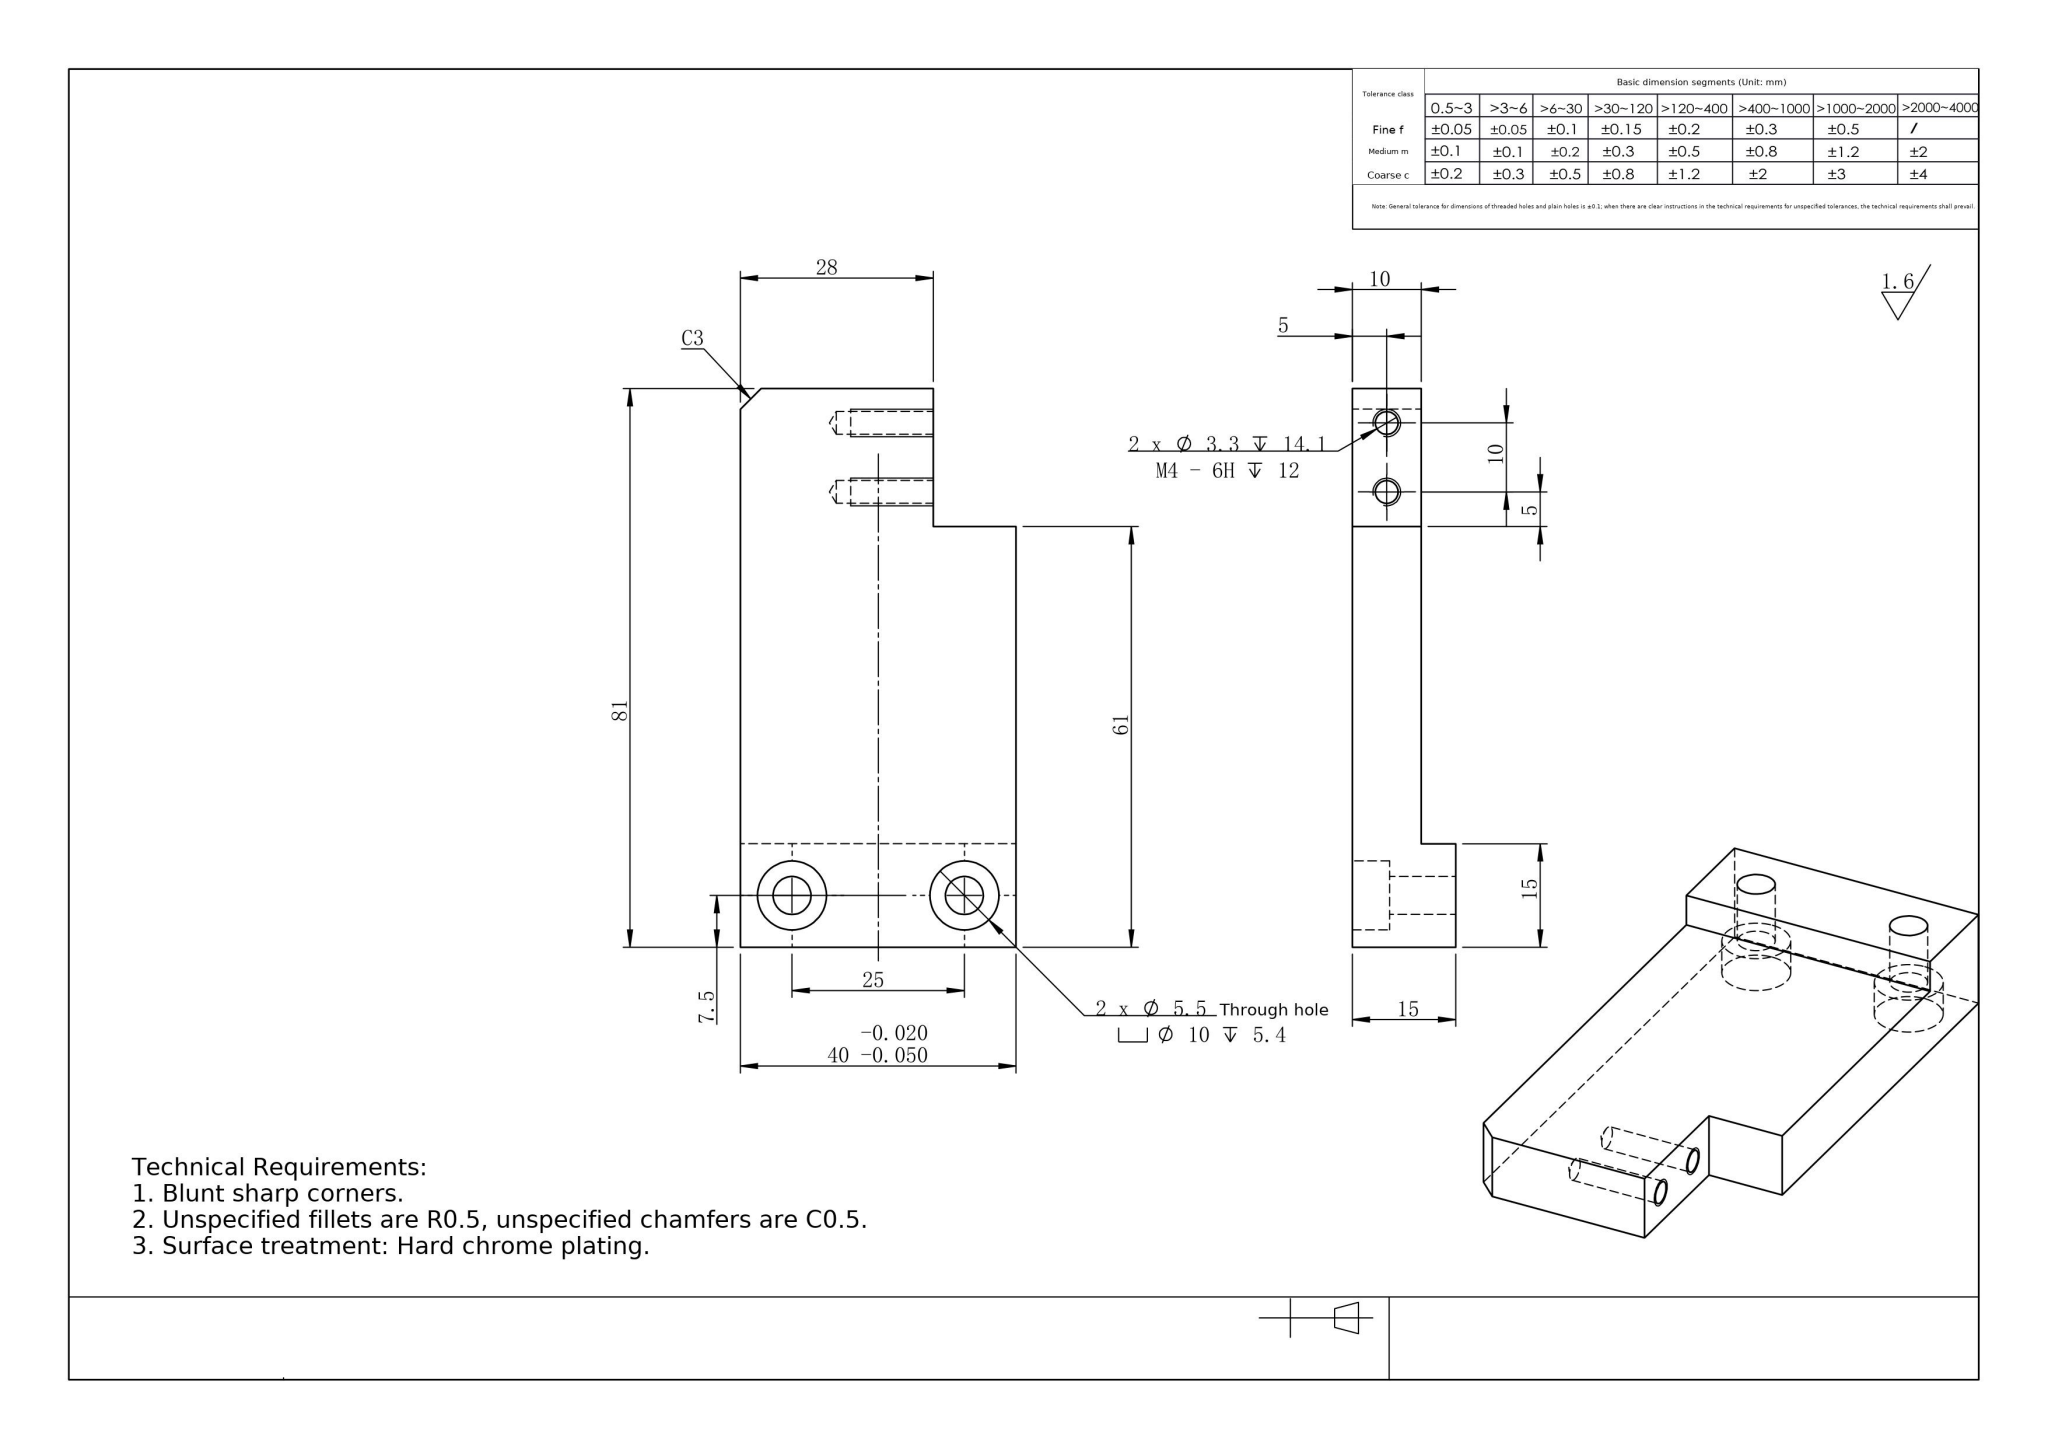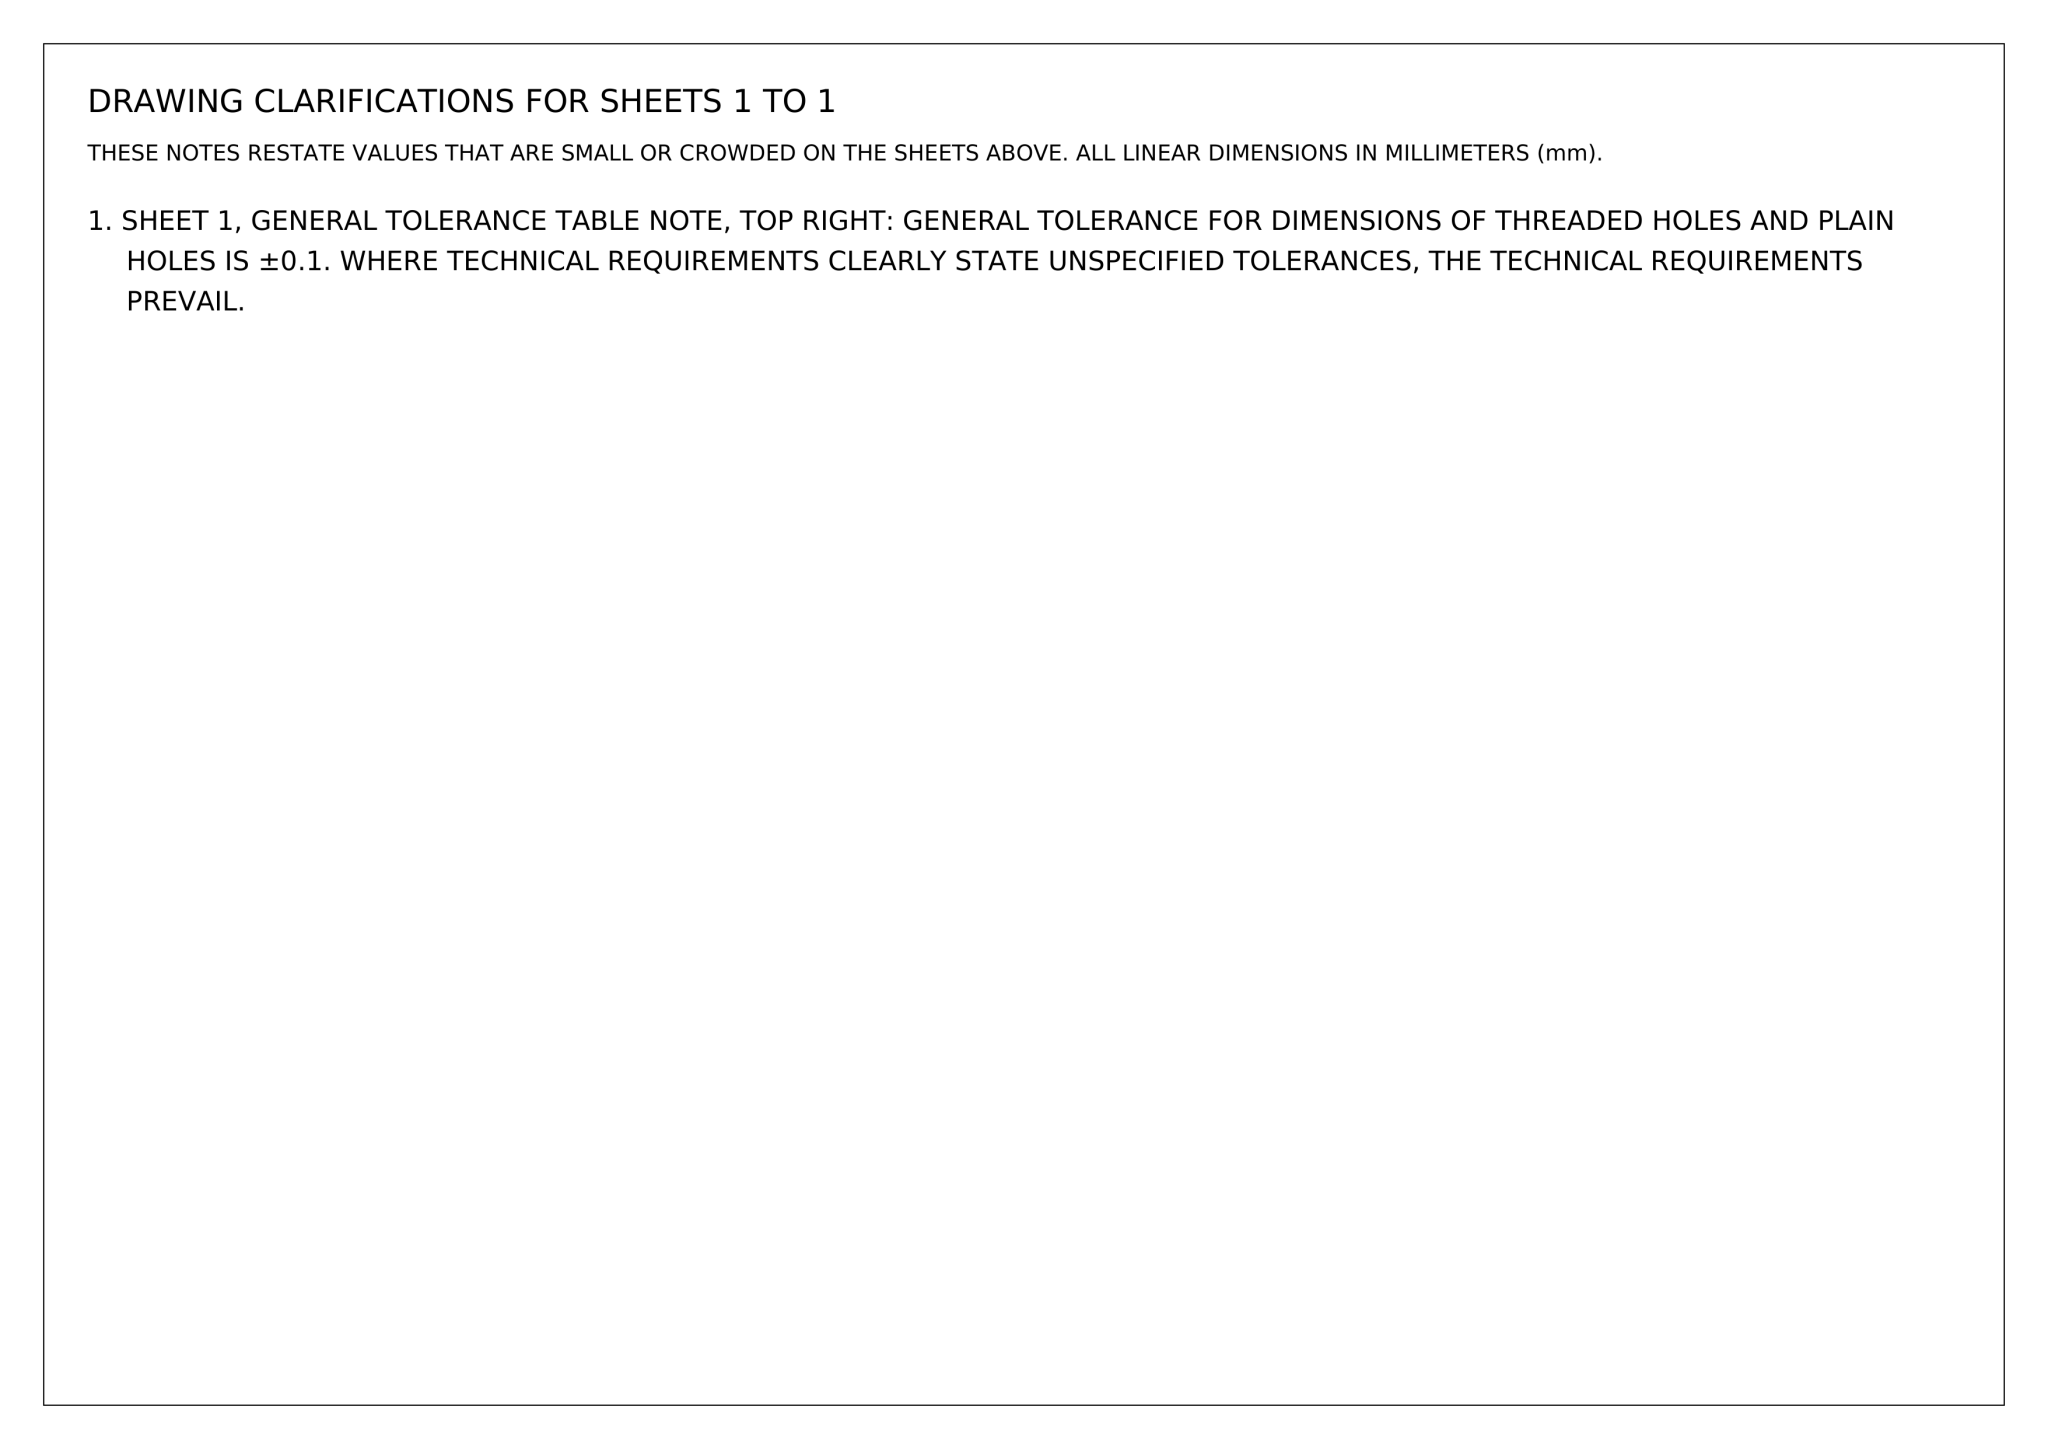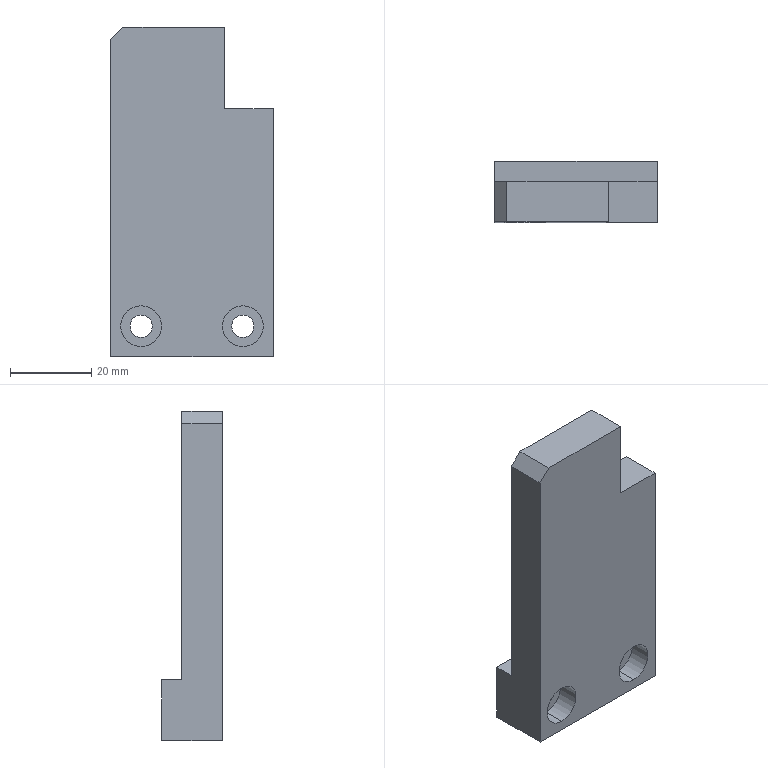Part | NX | mm | 1 solid | 29 faces | box 40 x 15 x 81 mm | volume 31404 mm3 | plane 13 | cylinder 12 | cone 4 | commonest cylinder face diameters 3.3 x4 10 x4 5.5 x4